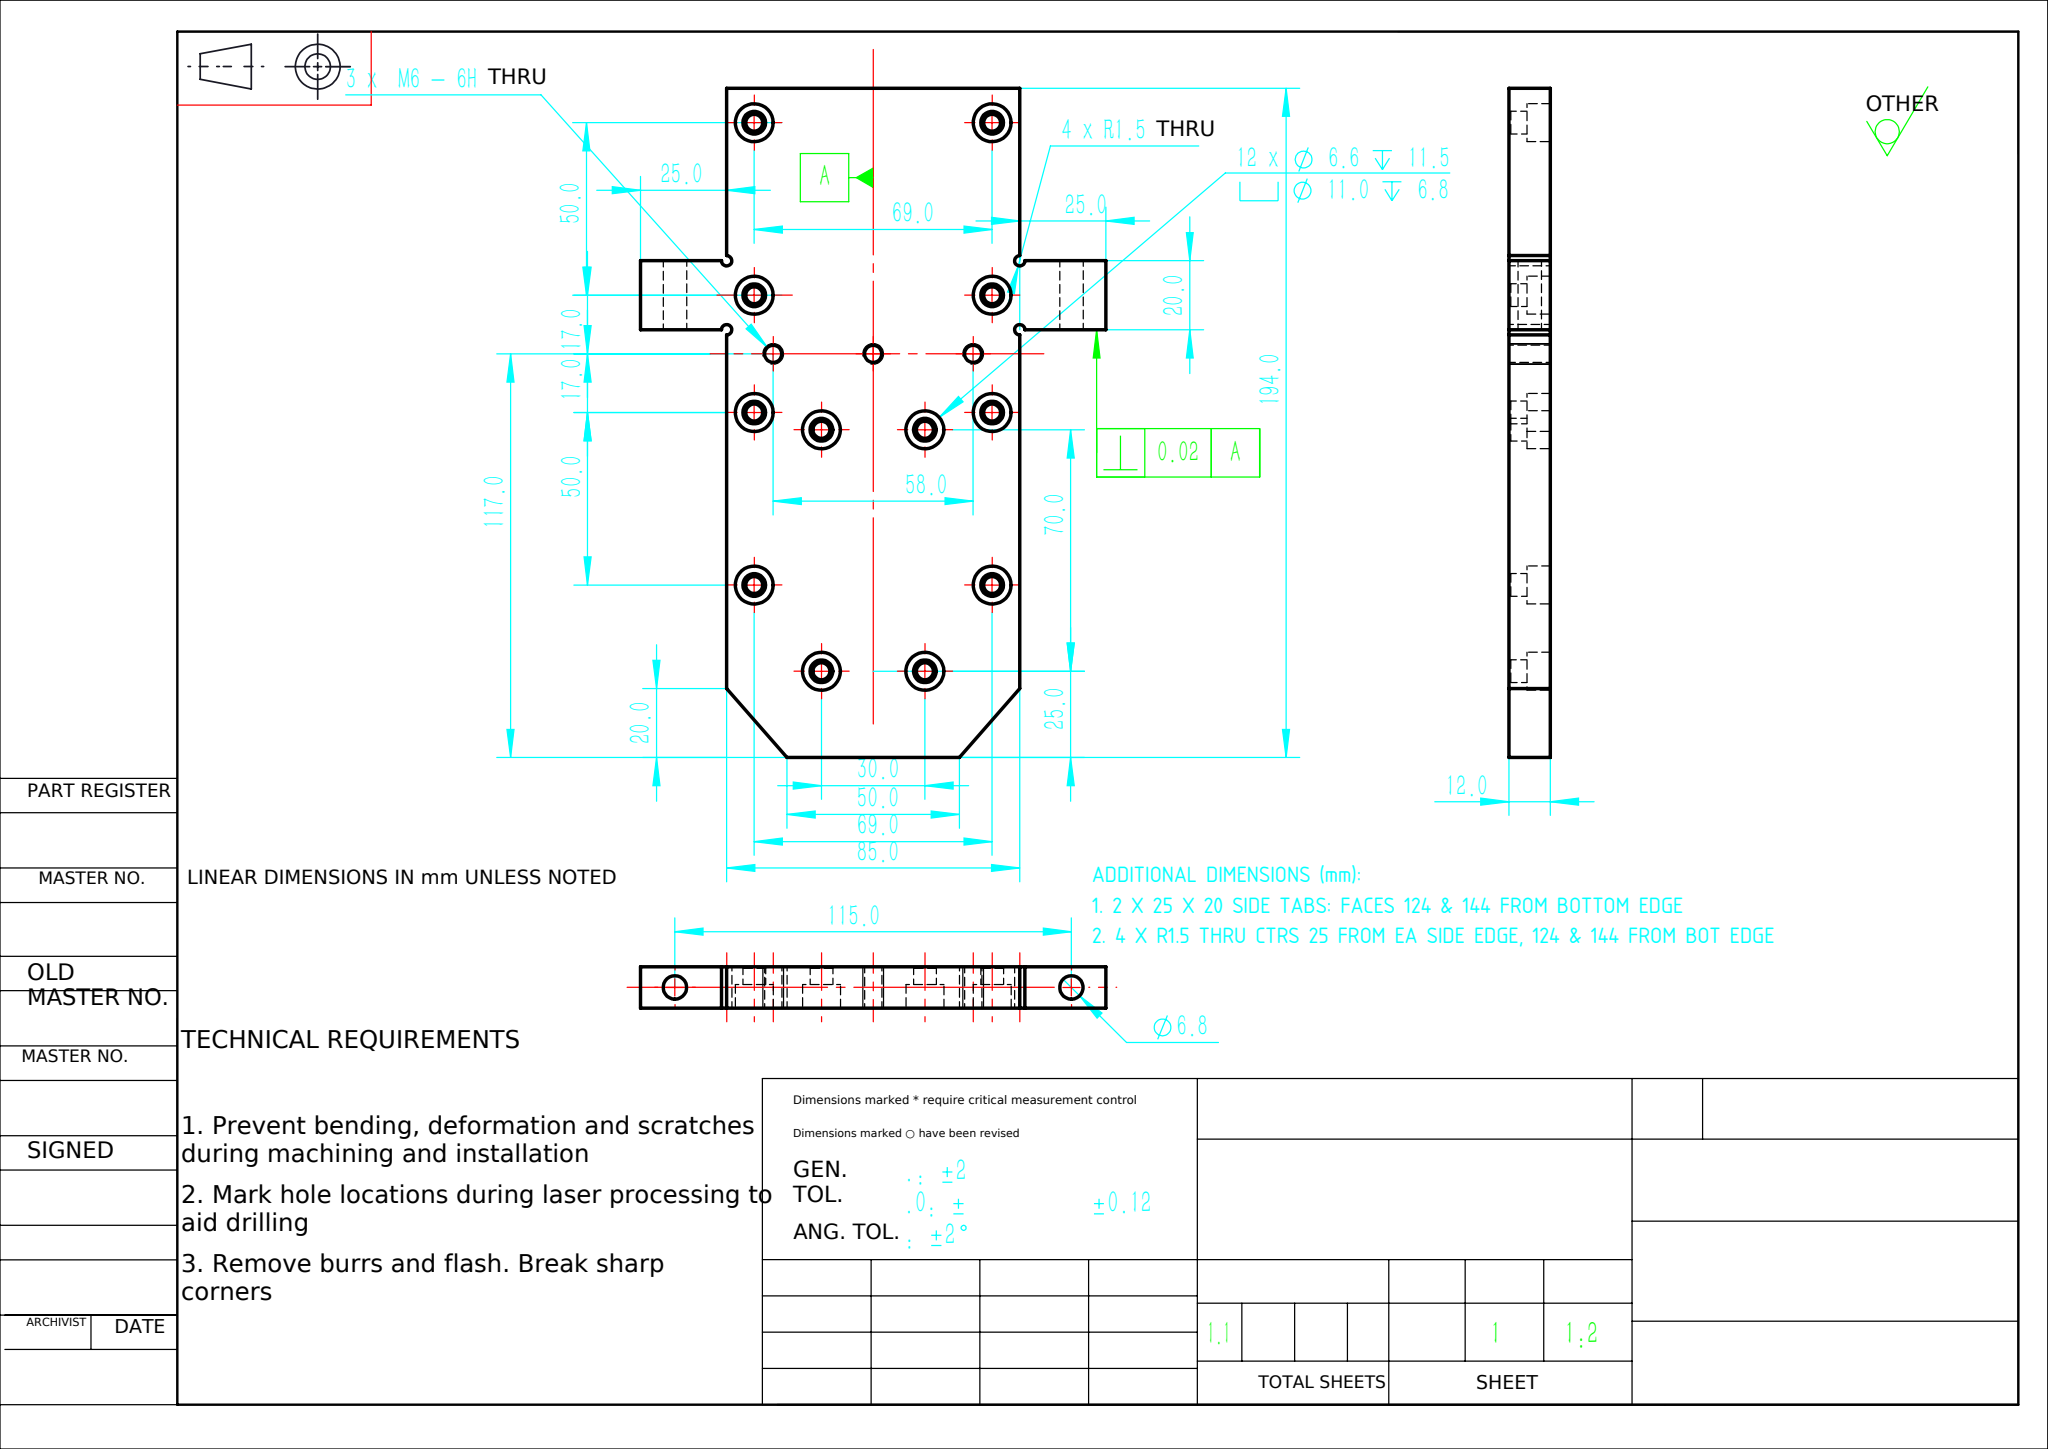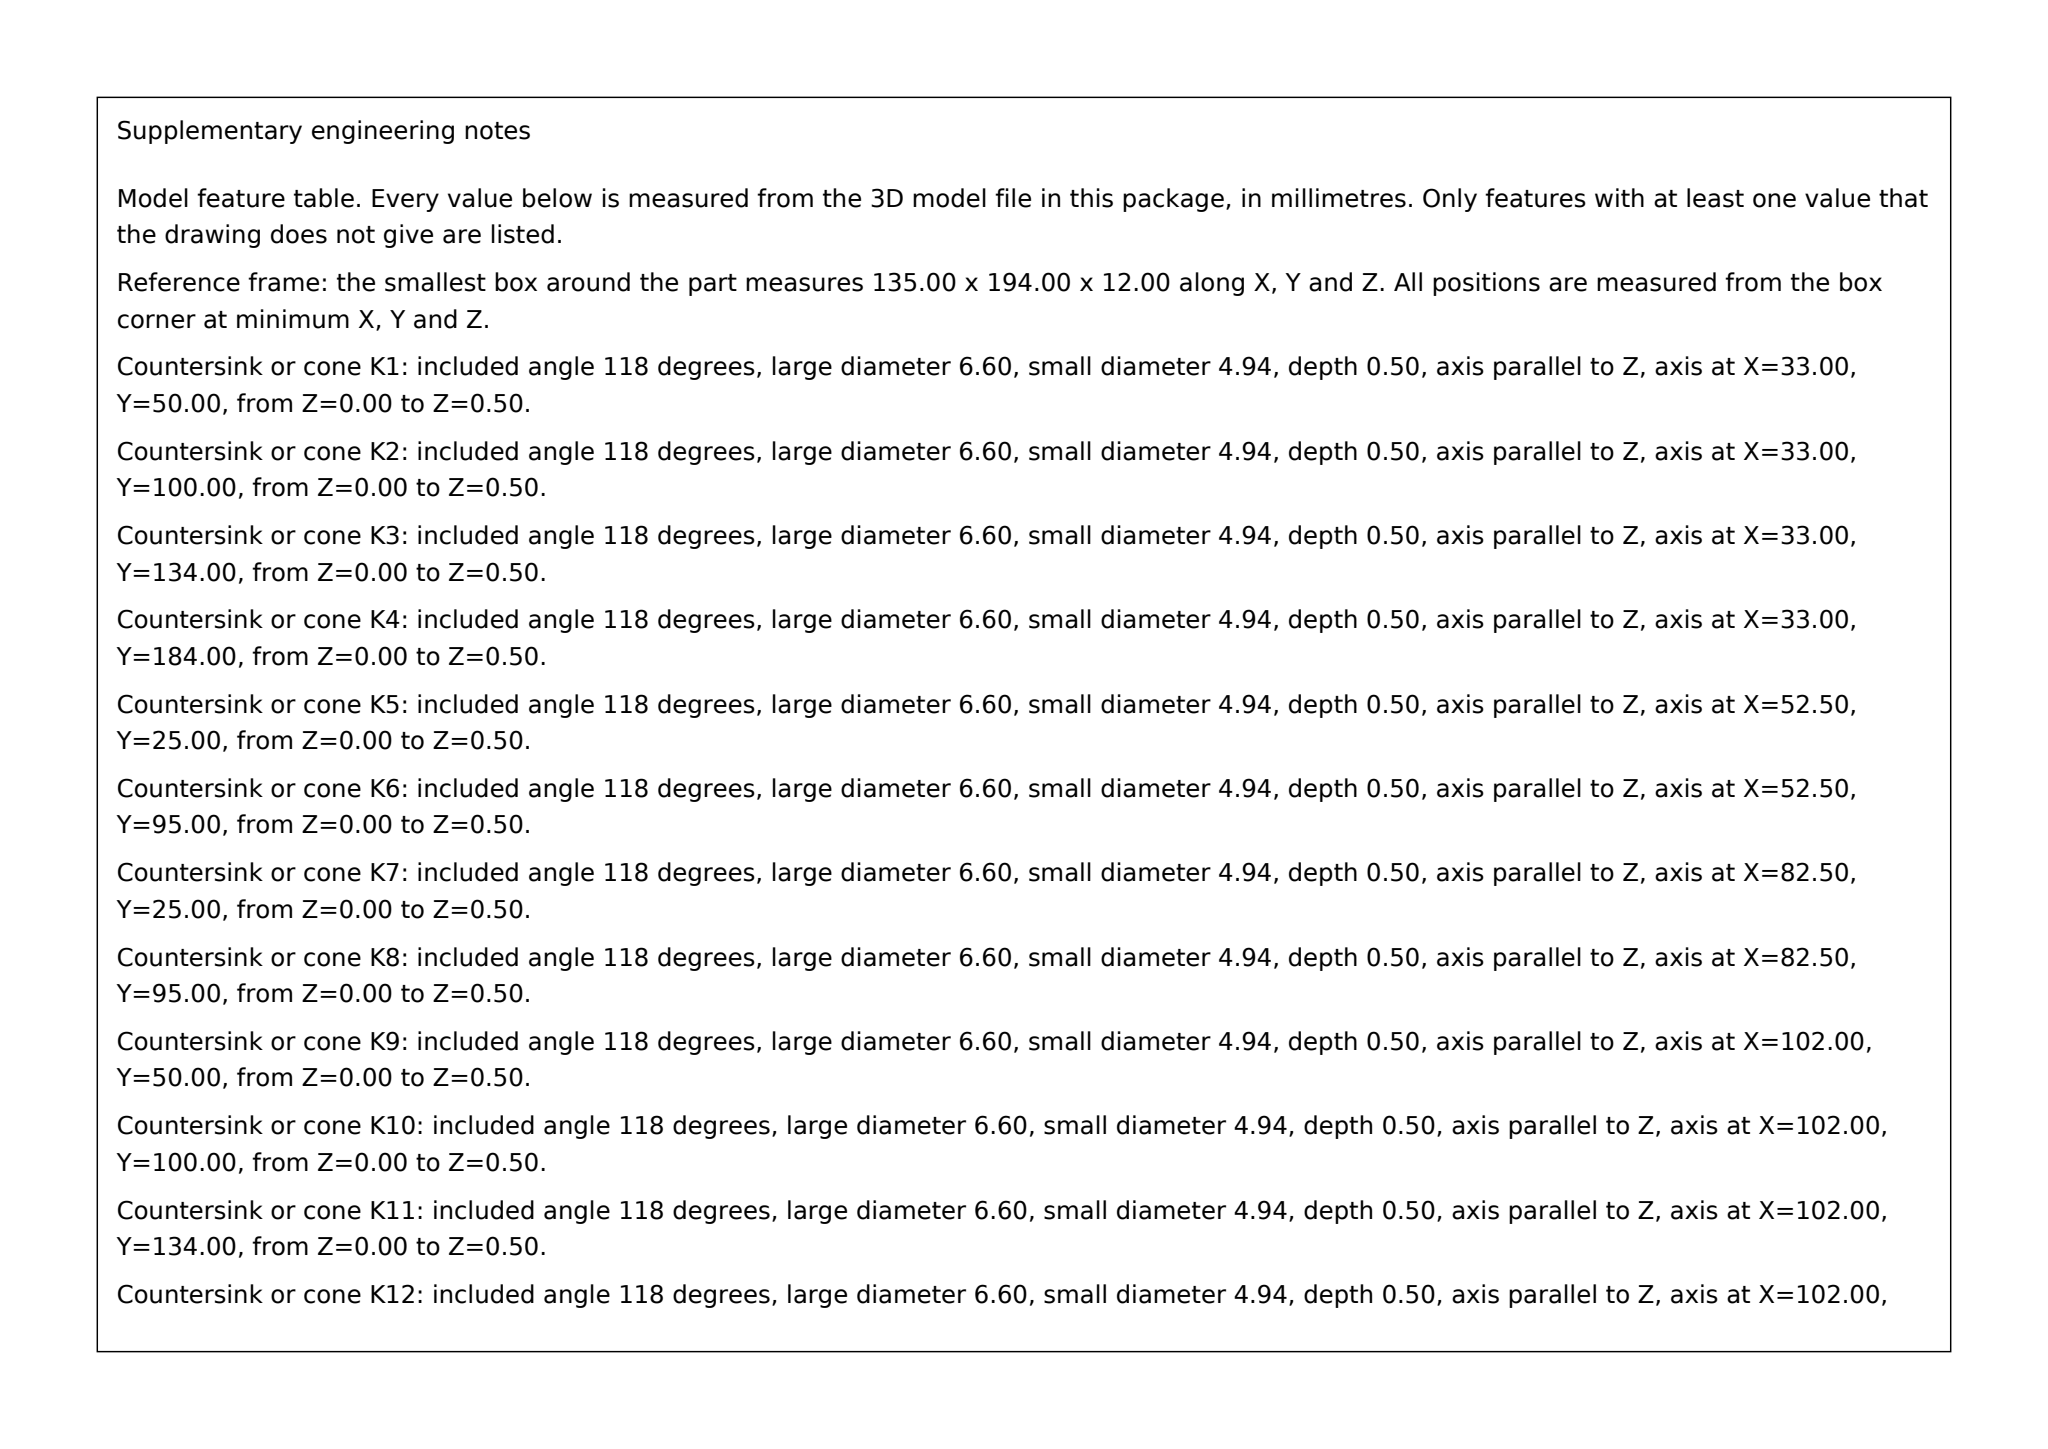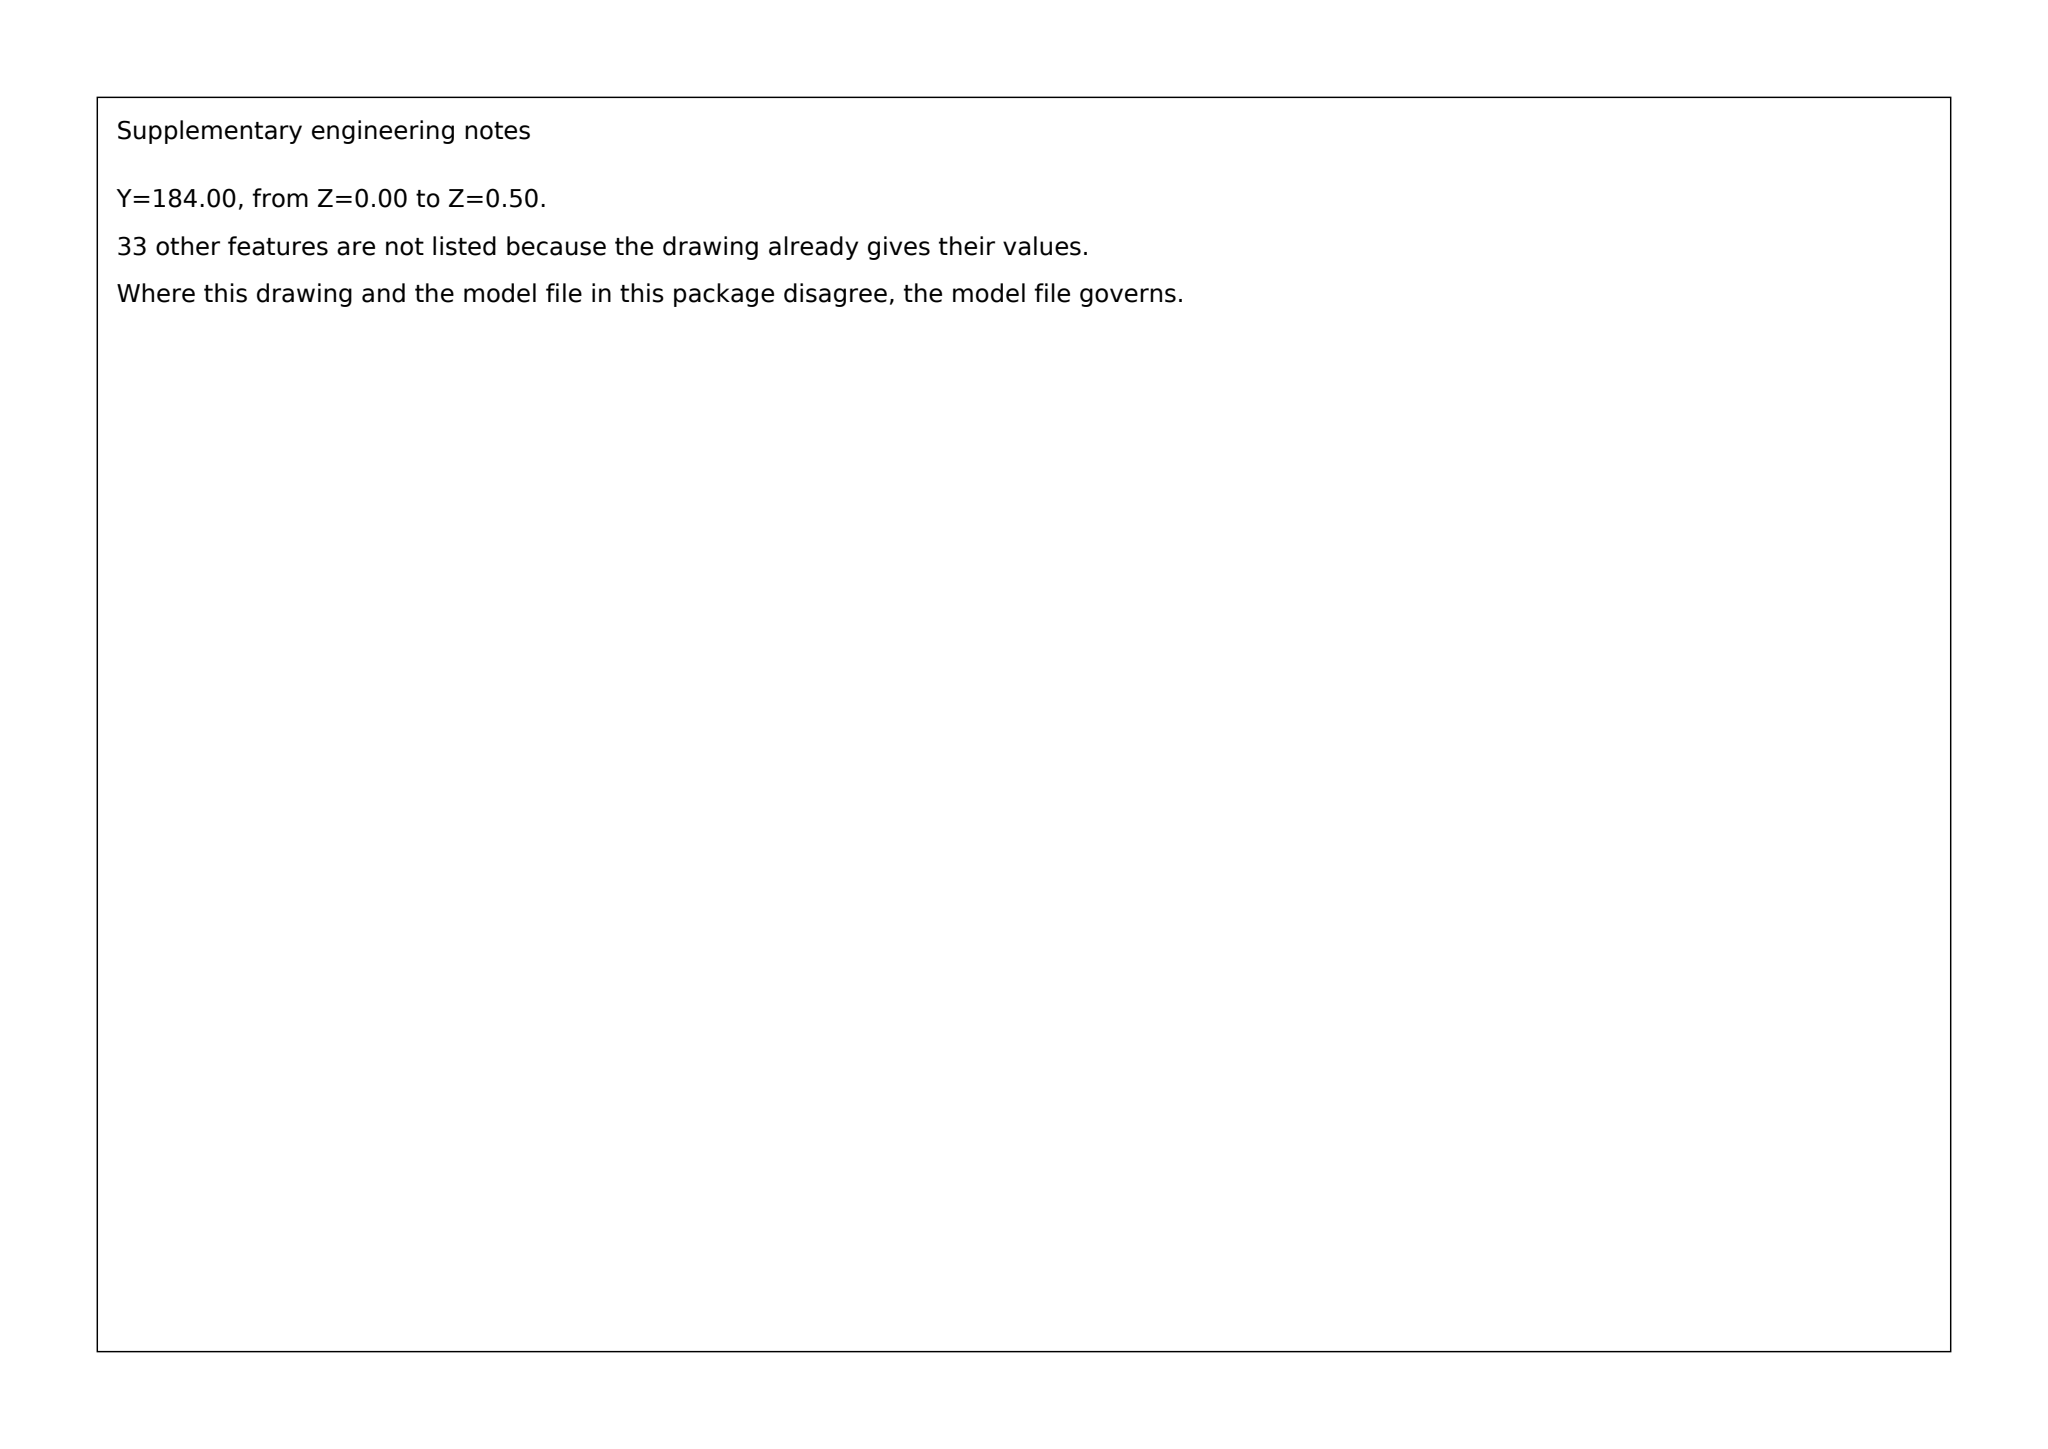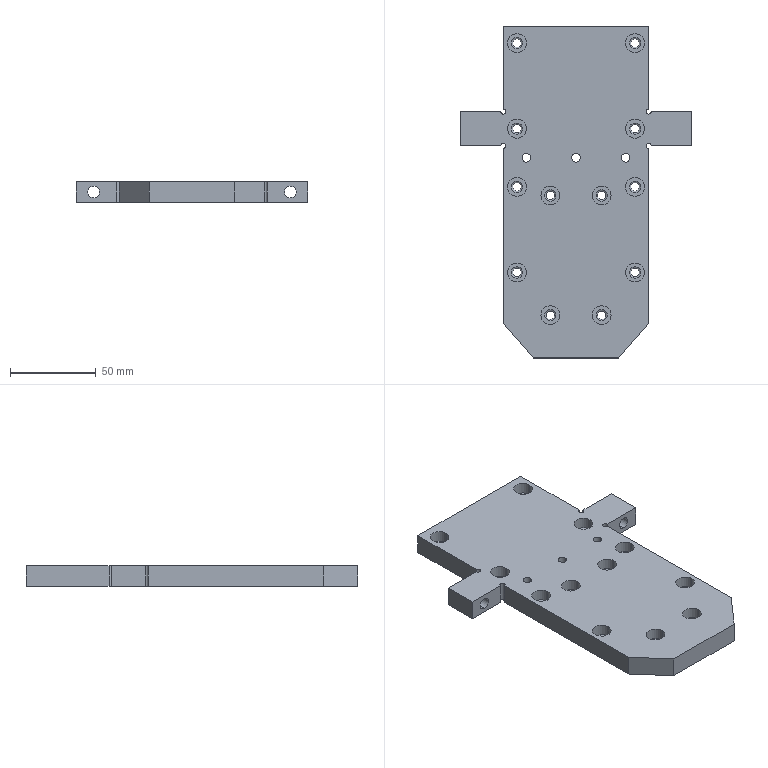Part | SolidWorks | mm | 1 solid | 116 faces | box 135 x 194 x 12 mm | volume 193424 mm3 | cylinder 64 | plane 28 | cone 24 | commonest cylinder face diameters 11 x24 6.6 x24 3 x6 5 x6 6.8 x4
build123d program:
from build123d import *

# Parameters (mm, degrees)
BOSS_EXTRUDE1_DEPTH                               = 12
HOLE_SIZE_ACCORDING_TO_TYPE_OF_HEXAGO_D           = 6.6
HOLE_SIZE_ACCORDING_TO_TYPE_OF_HEXAGO_DEPTH       = 11.5
HOLE_SIZE_ACCORDING_TO_TYPE_OF_HEXAGO_CBORE_D     = 11
HOLE_SIZE_ACCORDING_TO_TYPE_OF_HEXAGO_CBORE_DEPTH = 6.8
HOLE_SIZE_ACCORDING_TO_TYPE_OF_HEXAGO_TIP         = 1.983
M6_TAPPED_HOLE1_D                                 = 5
F_6_8_6_8_DIAMETER_HOLE1_D                        = 6.8
SKETCH9_R                                         = 1.5
CUT_EXTRUDE1_DEPTH                                = 40


with BuildPart() as part:
    # Sketch1 → Boss-Extrude1 (new body)
    with BuildSketch(Plane.XY):
        Polygon((7632.331, 2341.452), (7649.831, 2321.452), (7699.831, 2321.452), (7717.331, 2341.452), (7717.331, 2445.452), (7742.331, 2445.452), (7742.331, 2465.452), (7717.331, 2465.452), (7717.331, 2515.452), (7632.331, 2515.452), (7632.331, 2465.452), (7607.331, 2465.452), (7607.331, 2445.452), (7632.331, 2445.452), align=None)
    extrude(amount=BOSS_EXTRUDE1_DEPTH)

    # Hole Size _ according to_ Type of Hexago
    with Locations(Plane.XY.offset(12)):
        with Locations((7689.831, 2416.452), (7689.831, 2346.452), (7659.831, 2346.452), (7659.831, 2416.452), (7640.331, 2505.452), (7640.331, 2455.452), (7640.331, 2421.452), (7640.331, 2371.452), (7709.331, 2371.452), (7709.331, 2421.452), (7709.331, 2455.452), (7709.331, 2505.452)):
            CounterBoreHole(HOLE_SIZE_ACCORDING_TO_TYPE_OF_HEXAGO_D / 2, HOLE_SIZE_ACCORDING_TO_TYPE_OF_HEXAGO_CBORE_D / 2, HOLE_SIZE_ACCORDING_TO_TYPE_OF_HEXAGO_CBORE_DEPTH, depth=HOLE_SIZE_ACCORDING_TO_TYPE_OF_HEXAGO_DEPTH)
            with Locations((0, 0, -(HOLE_SIZE_ACCORDING_TO_TYPE_OF_HEXAGO_DEPTH + HOLE_SIZE_ACCORDING_TO_TYPE_OF_HEXAGO_TIP / 2))):  # 118° drill point
                Cone(0, HOLE_SIZE_ACCORDING_TO_TYPE_OF_HEXAGO_D / 2, HOLE_SIZE_ACCORDING_TO_TYPE_OF_HEXAGO_TIP, mode=Mode.SUBTRACT)

    # M6 Tapped Hole1 (through all)
    with Locations(Plane.XY.offset(12)):
        with Locations((7645.831, 2438.452), (7674.831, 2438.452), (7703.831, 2438.452)):
            Hole(M6_TAPPED_HOLE1_D / 2)

    # 6.8 _6.8_ Diameter Hole1 (through all)
    with Locations(Plane(origin=(0, 2465.452, 0), x_dir=(1, 0, 0), z_dir=(0, 1, 0))):
        with Locations((7732.331, -6), (7617.331, -6)):
            Hole(F_6_8_6_8_DIAMETER_HOLE1_D / 2)

    # Sketch9 → Cut-Extrude1 (cut)
    with BuildSketch(Plane.XY.offset(12)):
        with Locations((7717.331, 2465.452)):
            Circle(SKETCH9_R)
        with Locations((7717.331, 2445.452)):
            Circle(SKETCH9_R)
        with Locations((7632.331, 2445.452)):
            Circle(SKETCH9_R)
        with Locations((7632.331, 2465.452)):
            Circle(SKETCH9_R)
    extrude(amount=-CUT_EXTRUDE1_DEPTH, mode=Mode.SUBTRACT)


solid = part.part